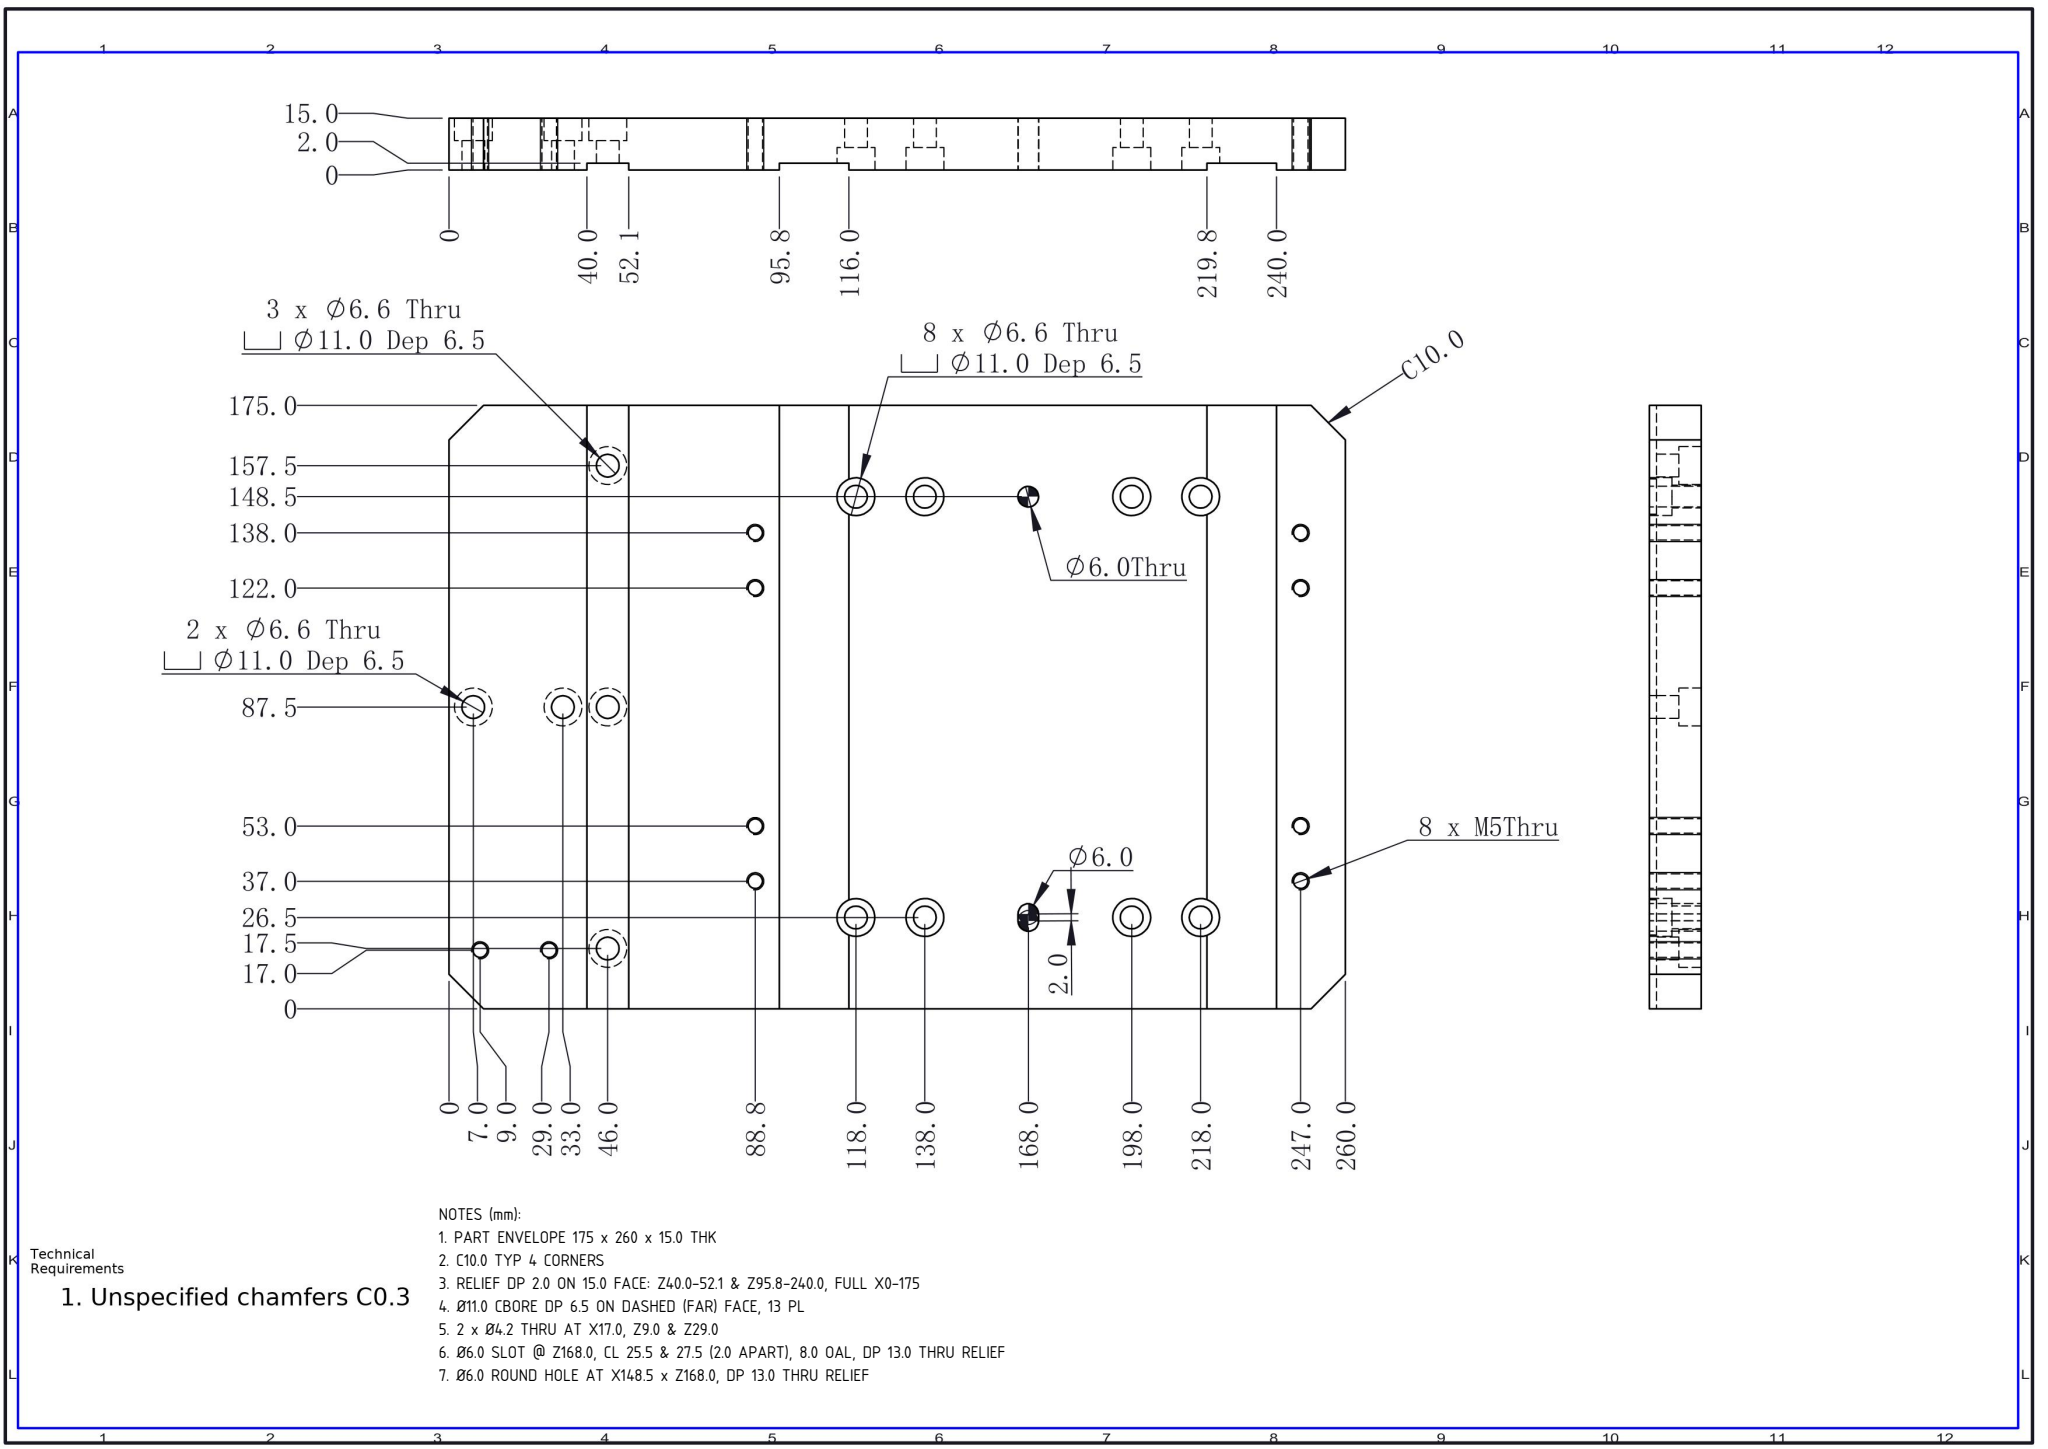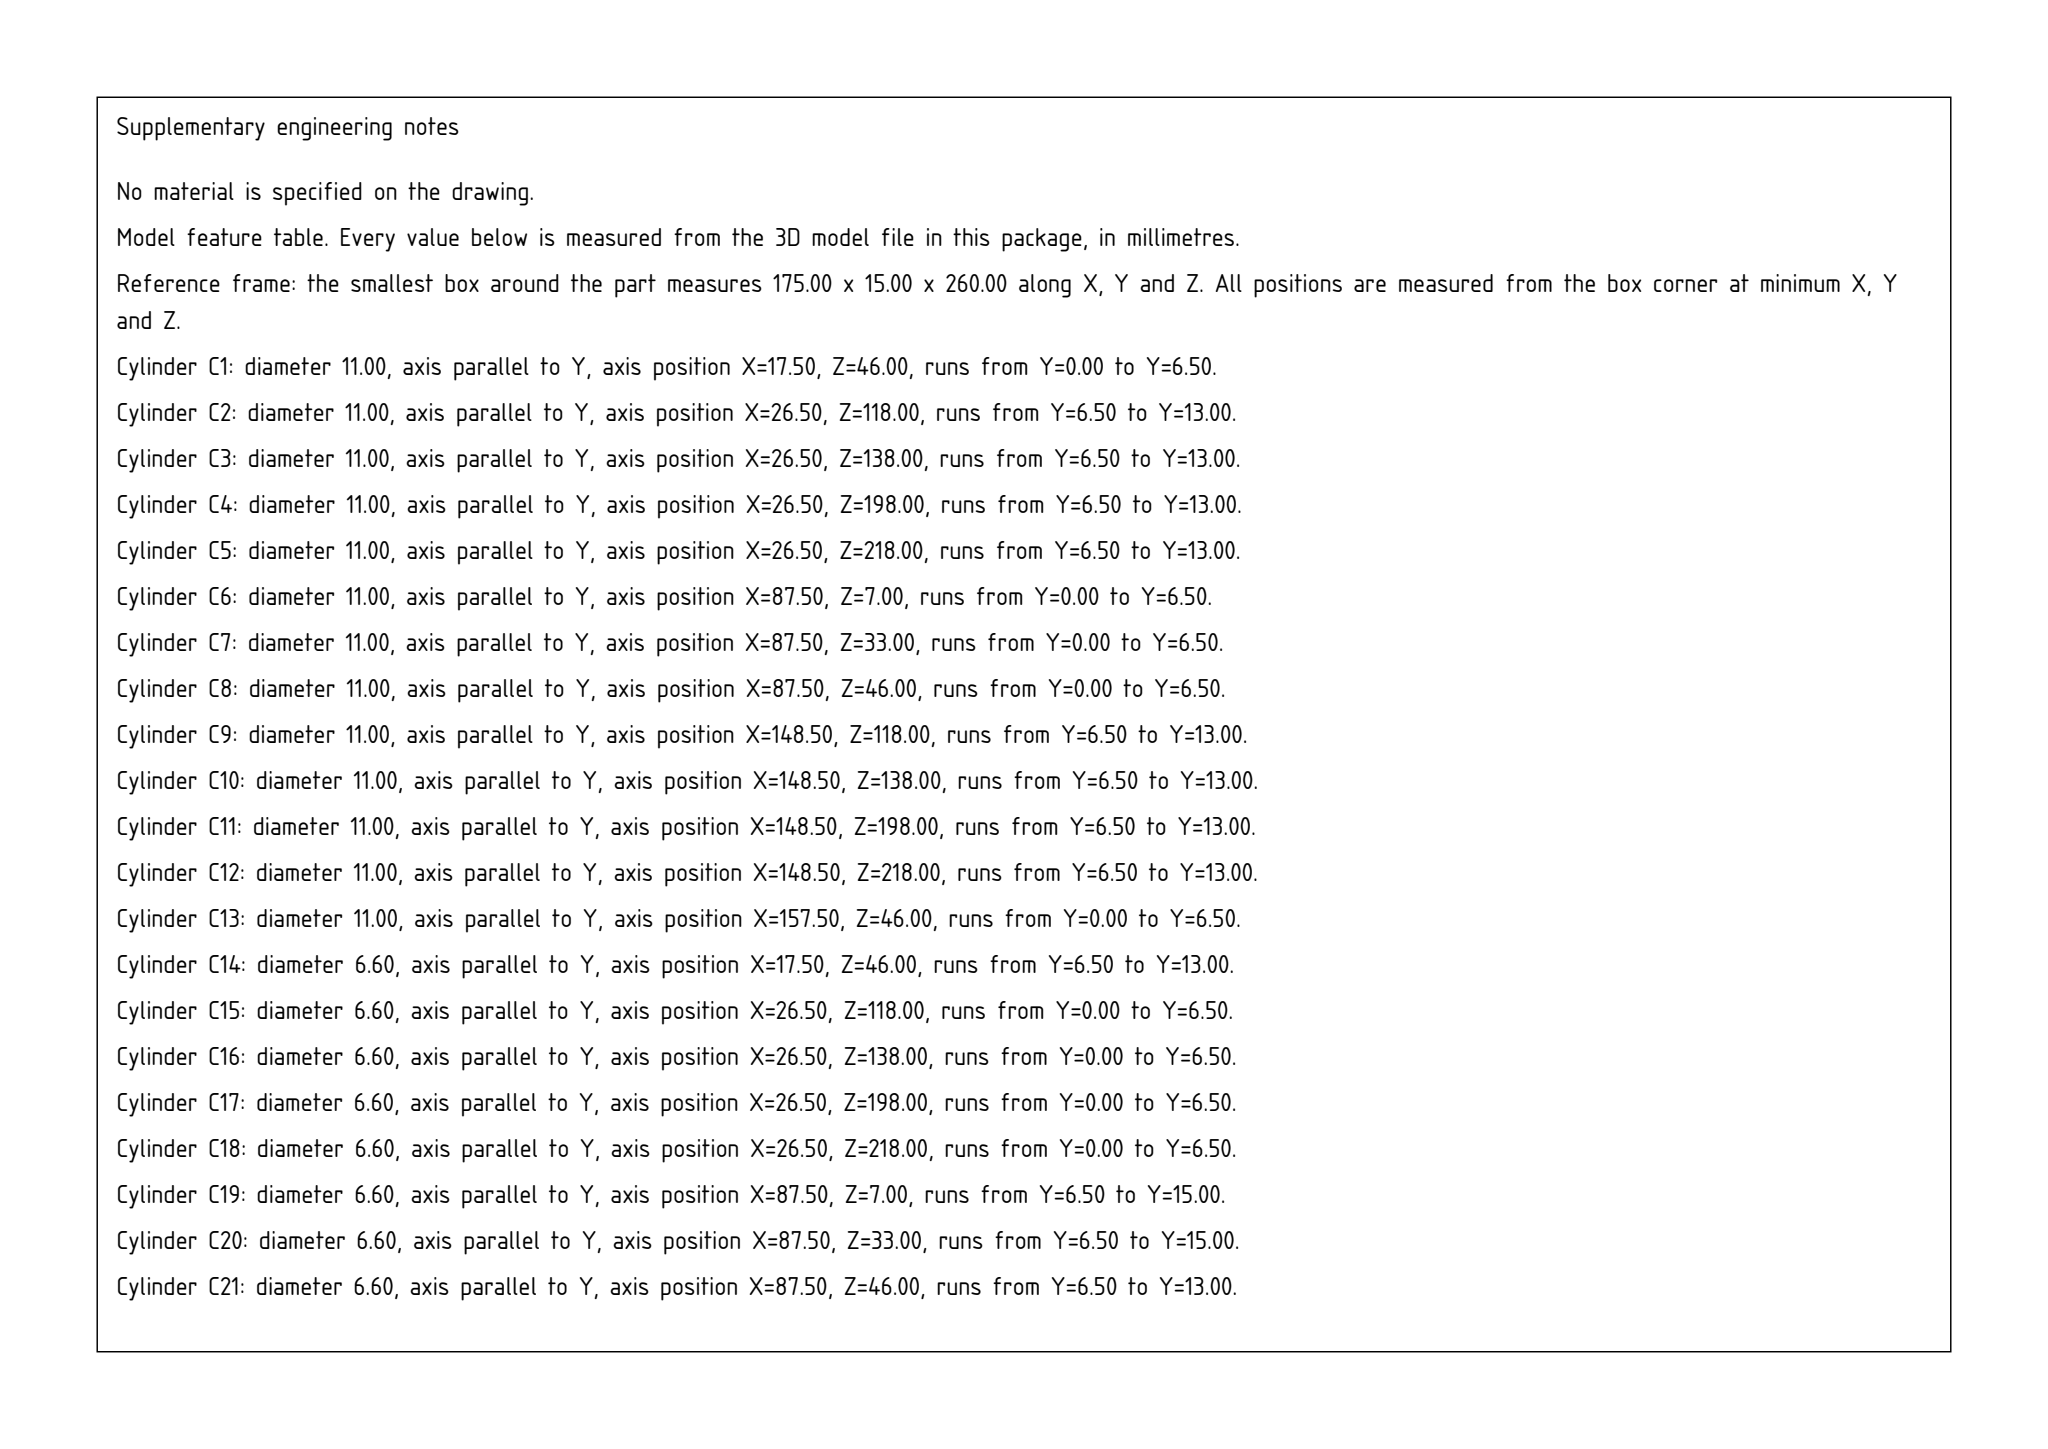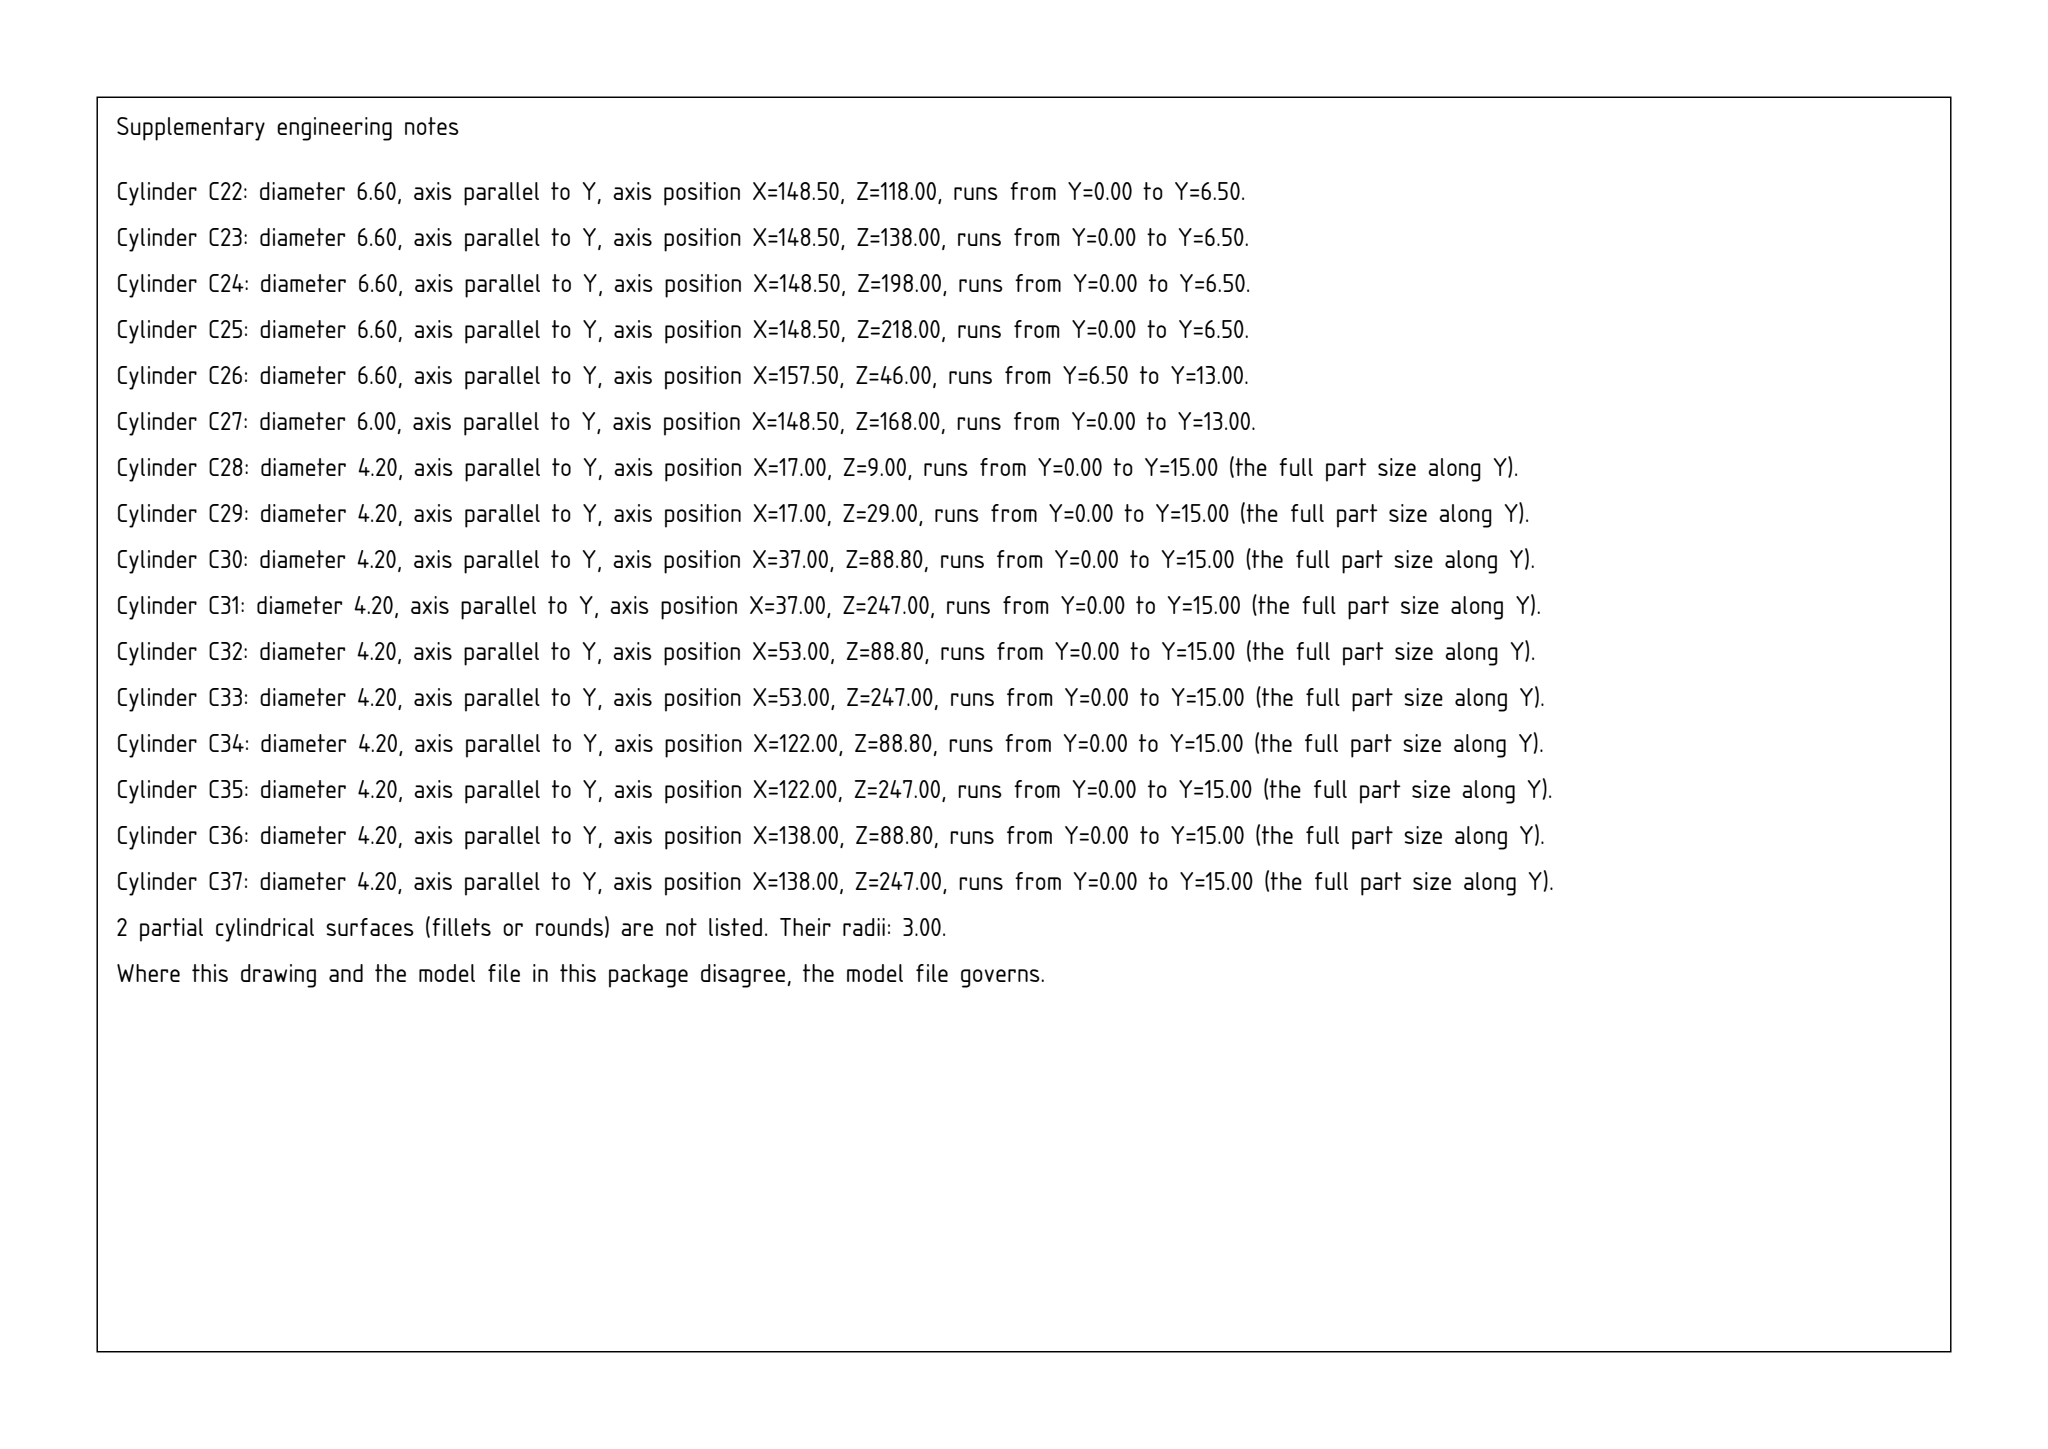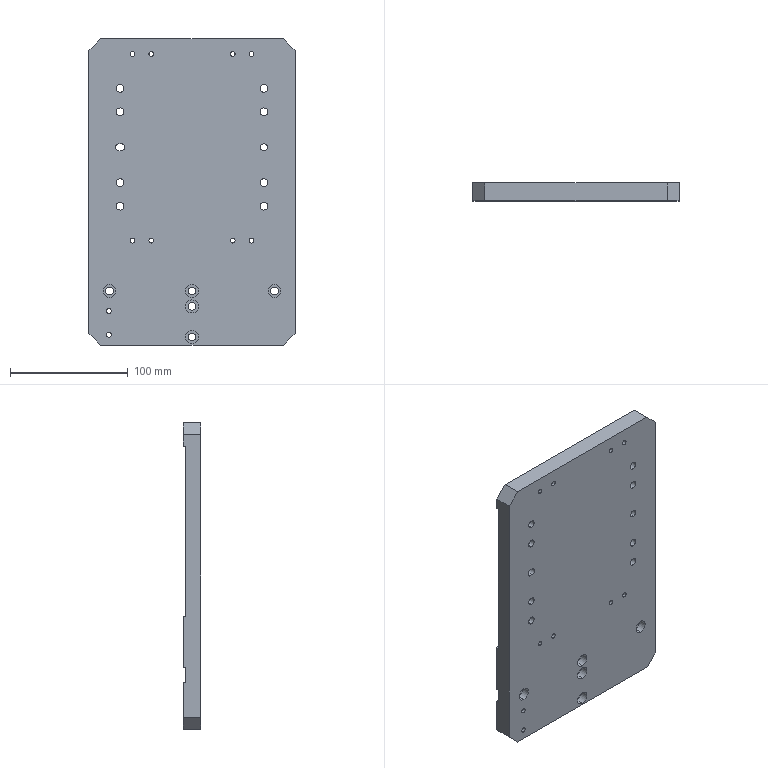Part | SolidWorks | mm | 1 solid | 110 faces | box 175 x 15 x 260 mm | volume 610768 mm3 | cylinder 77 | plane 33 | commonest cylinder face diameters 11 x26 6.6 x26 4.2 x20 6 x5
Drawing notes:
PART ENVELOPE 175 x 260 x 15.0 THK | from the solid: bbox_xyz 175.0 x 15.0 x 260.0; y-planes 0.0 and 15.0
C10.0 TYP 4 CORNERS | from the solid: bbox 175x260 with 4 non-orthogonal corner chamfer faces; only x=0/175 & z=0/260 planes
RELIEF DP 2.0 ON 15.0 FACE: Z40.0-52.1 & Z95.8-240.0, FULL X0-175 | from the solid: z-planes 40.0/52.1/95.8/240.0; relief floor y=13.0 (15.0-2.0) bounded only by x=0 and x=175
Ø11.0 CBORE DP 6.5 ON DASHED (FAR) FACE, 13 PL | from the solid: 13 cylinders dia 11.0 axis y len 6.5, plus 13 y-planes at offset 6.5 = cbore floors
2 x Ø4.2 THRU AT X17.0, Z9.0 & Z29.0 | from the solid: dia 4.2 cyl axis y at [17.0,9.0] & [17.0,29.0], len 15.0 = thru
Ø6.0 SLOT @ Z168.0, CL 25.5 & 27.5 (2.0 APART), 8.0 OAL, DP 13.0 THRU RELIEF | from the solid: dia 6.0 cyls at [25.5,168.0] and [27.5,168.0], axis y, len 13.0
Ø6.0 ROUND HOLE AT X148.5 x Z168.0, DP 13.0 THRU RELIEF | from the solid: dia 6.0 cyl at [148.5,168.0], axis y, len 13.0, single CL